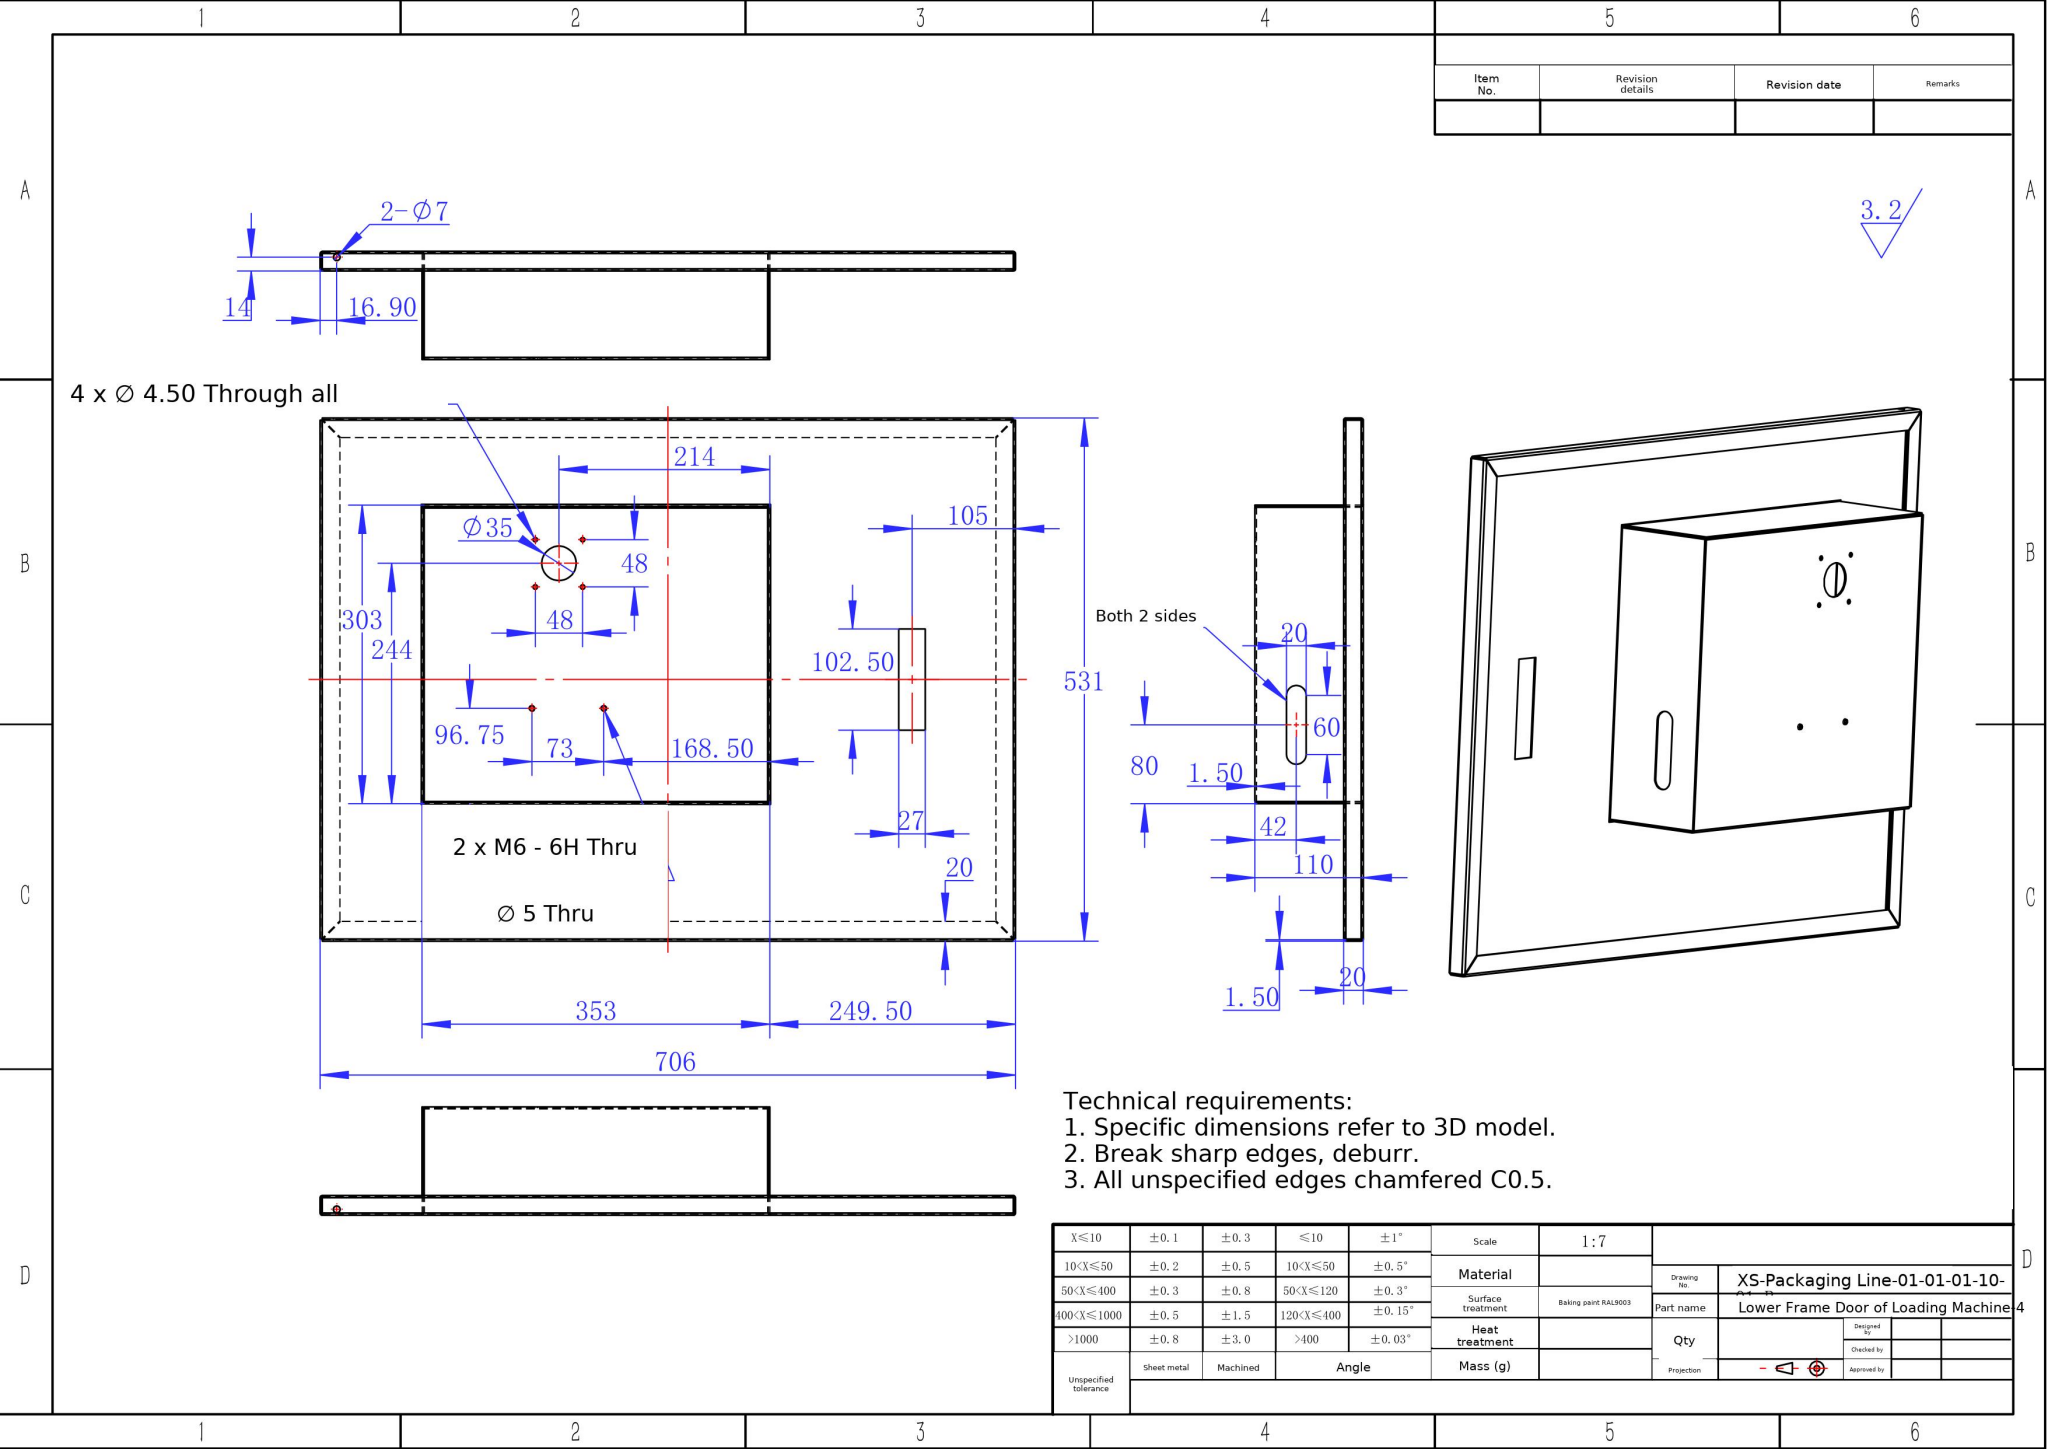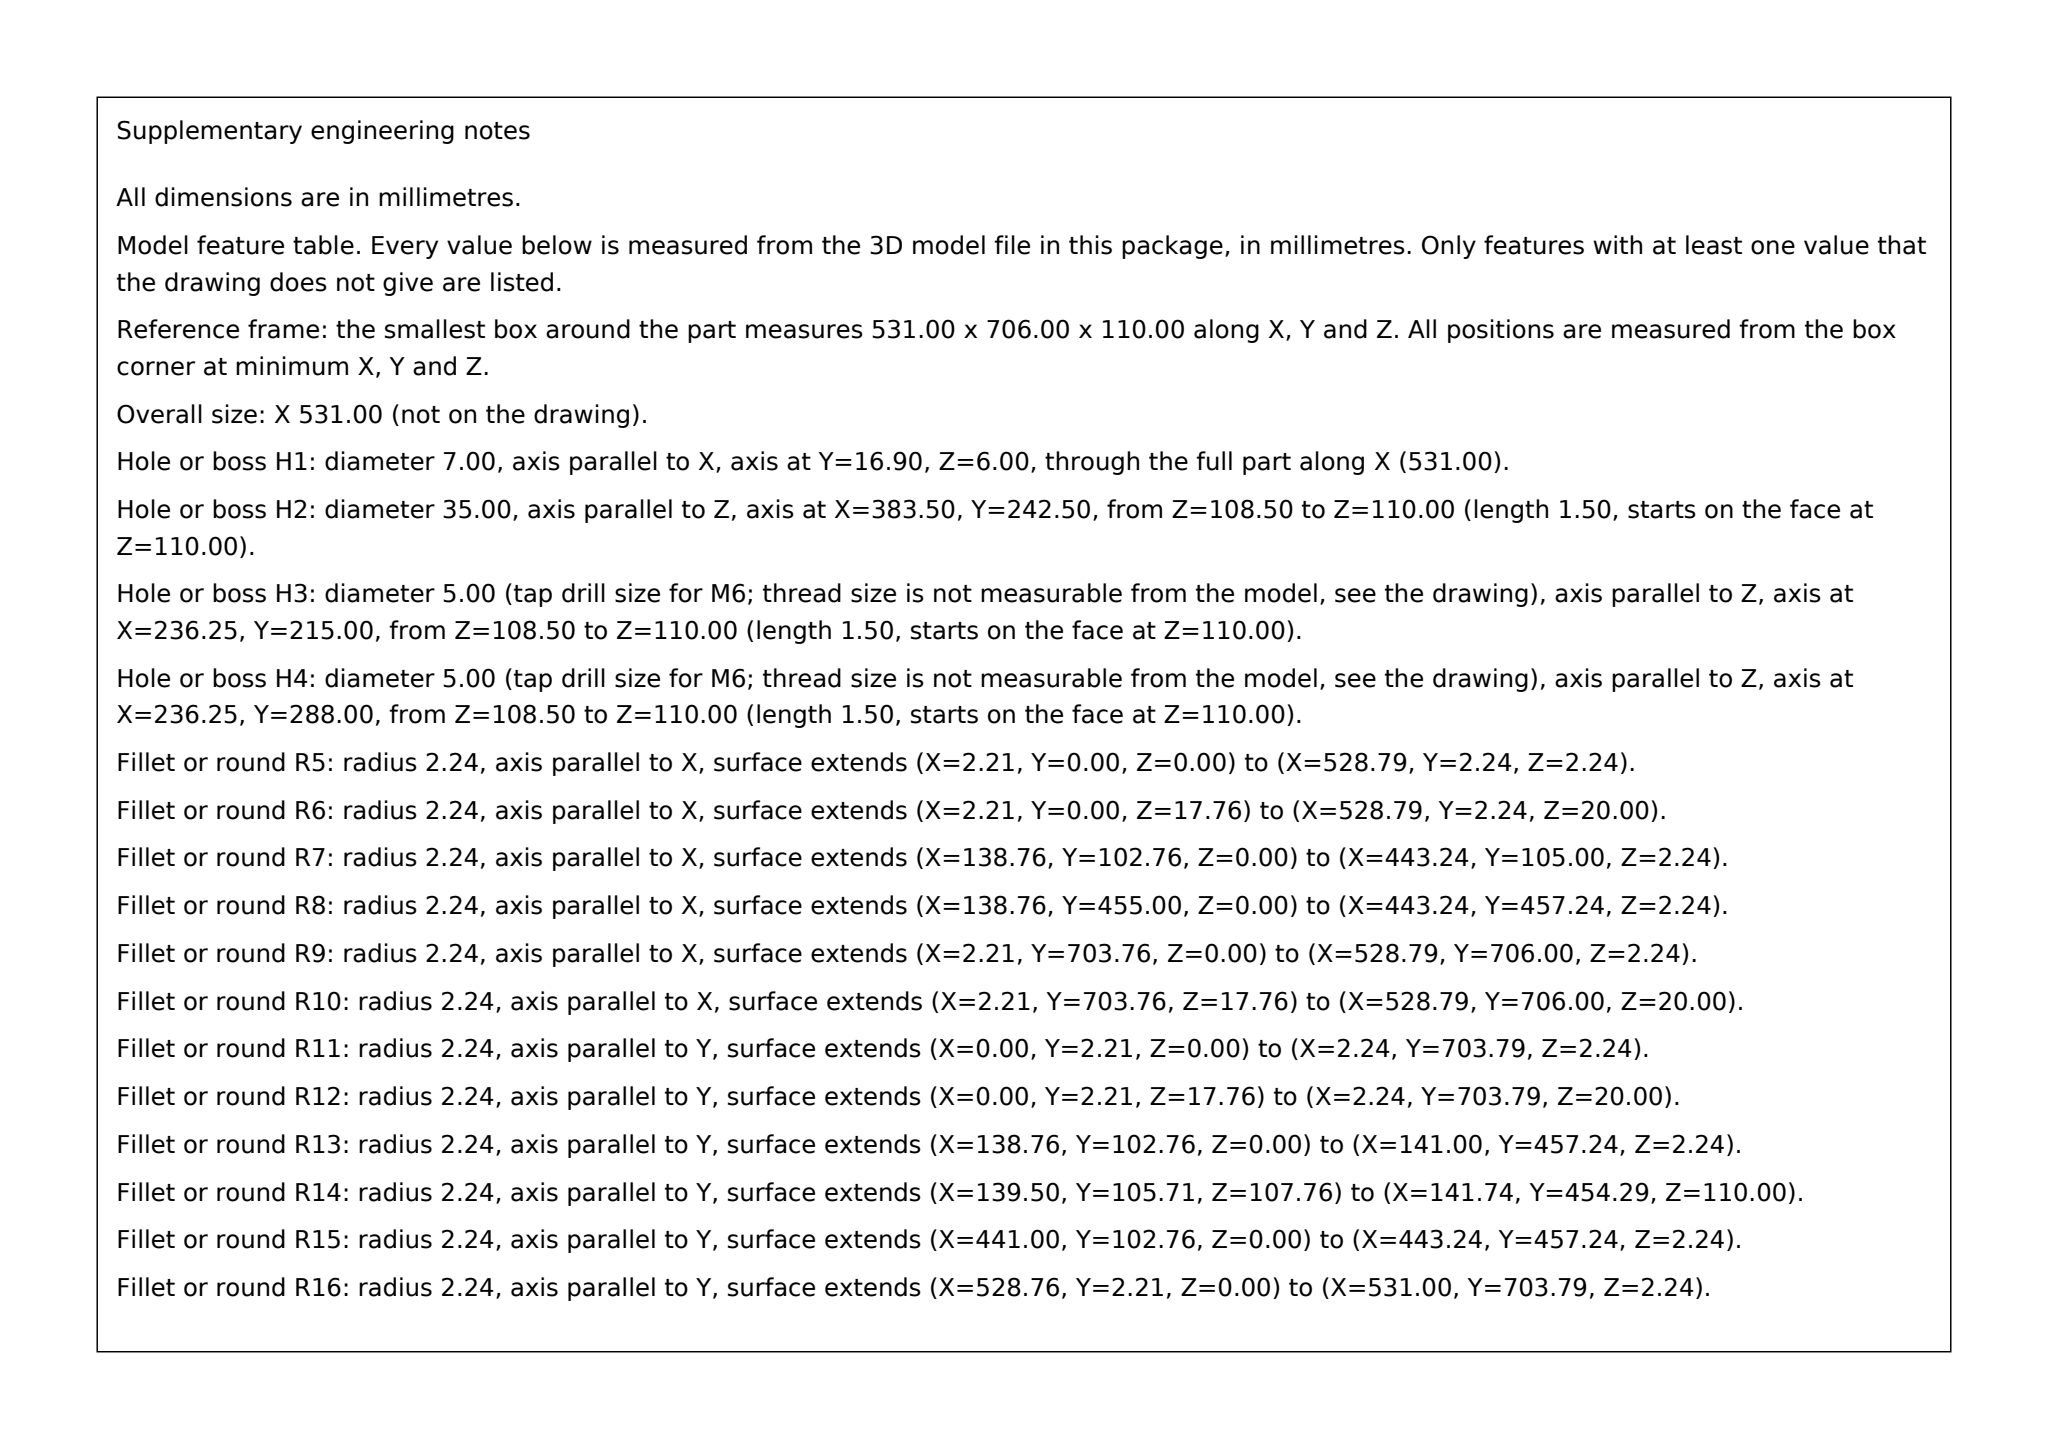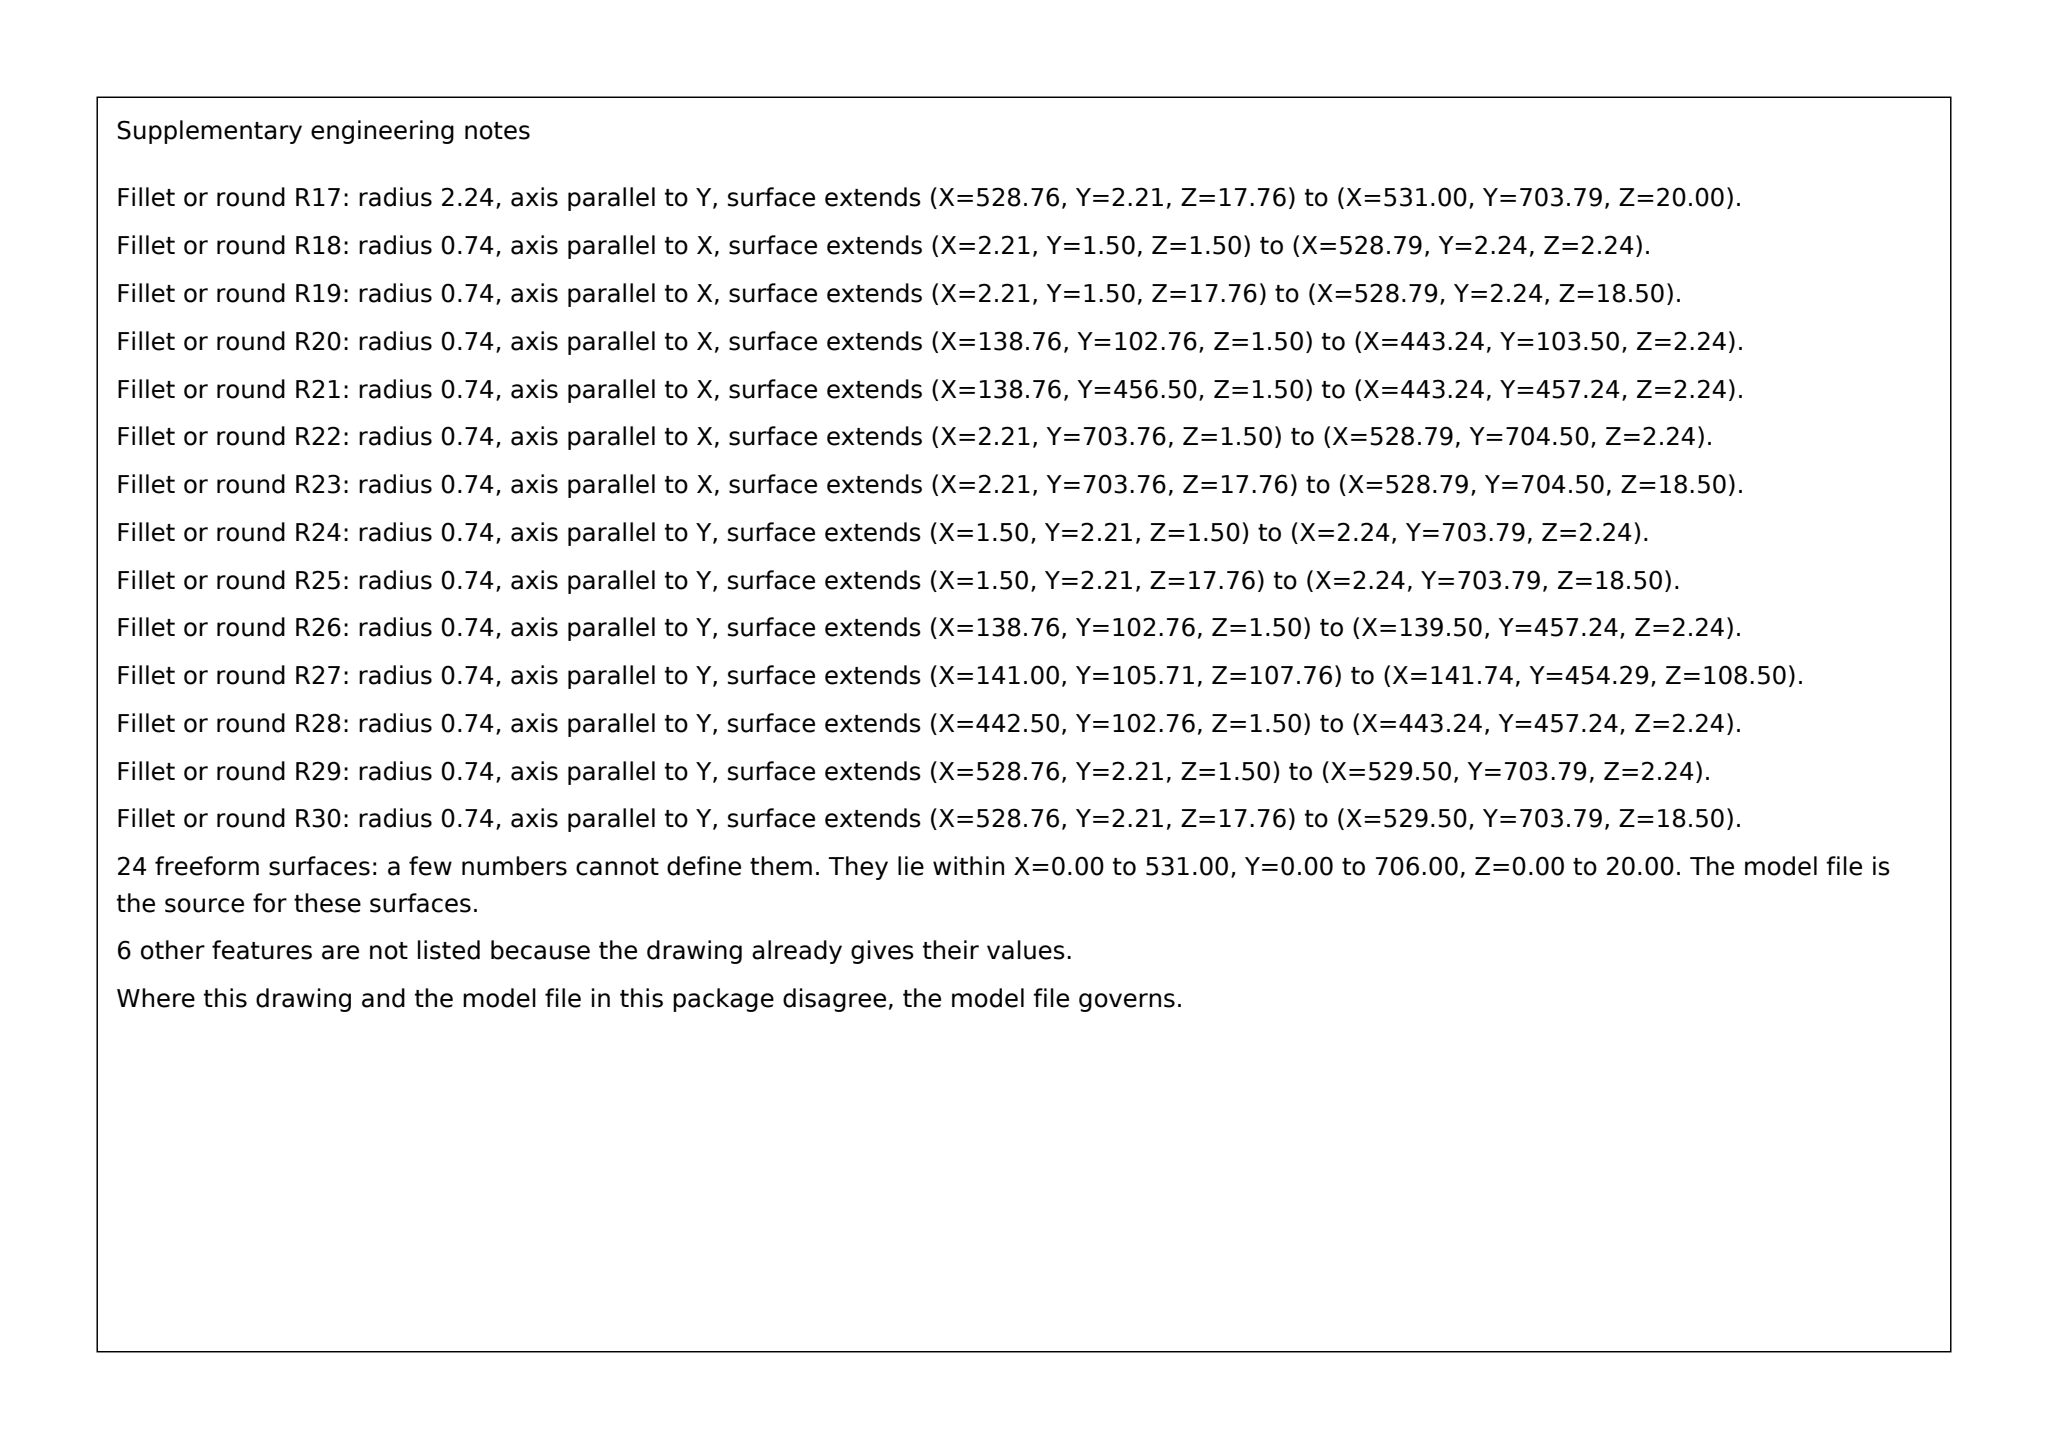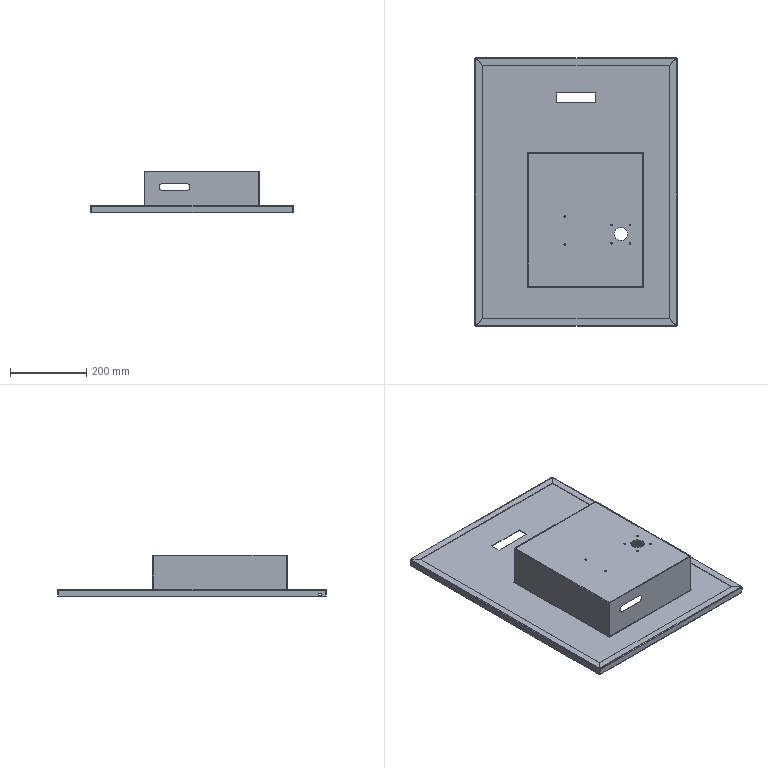Part | SolidWorks | mm | 1 solid | 144 faces | box 531 x 706 x 110 mm | volume 889111 mm3 | plane 72 | cylinder 48 | spline 24 | commonest cylinder face diameters 4.473 x13 1.473 x13 4.5 x8 5 x4 7 x4 20 x4 35 x2